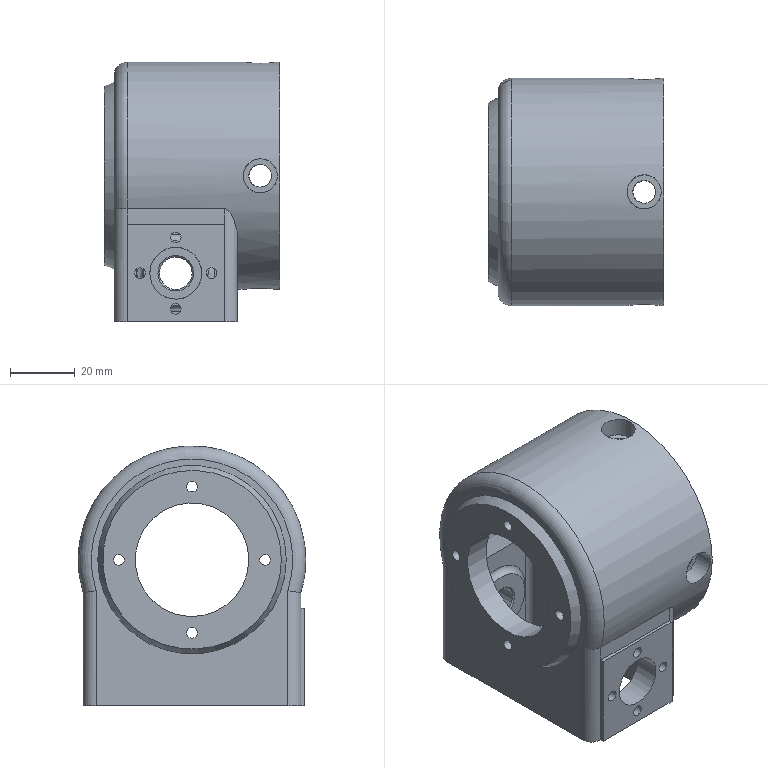Component | NX | GEARBOX | 1 solid | 61 faces | volume 86512 mm3 | cylinder 32 | plane 21 | torus 4 | cone 2 | spline 2 | commonest cylinder face diameters 3.3 x8 4 x6 7 x4 10.5 x4 8 x4 70 x1 55 x1 58 x1